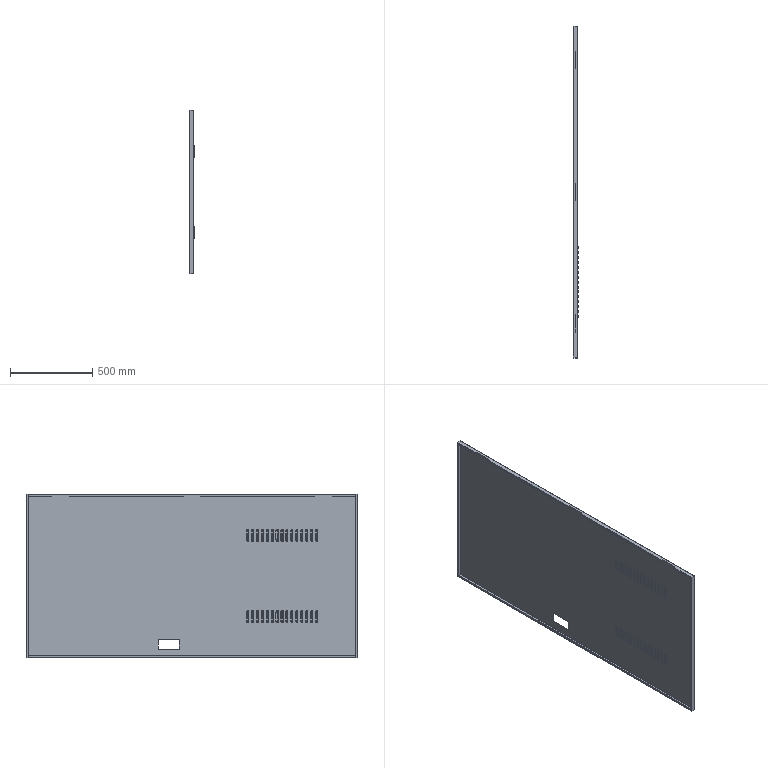Component | SolidWorks | SideDoorPanel-1 | 1 solid | 836 faces | volume 3311563 mm3 | cylinder 382 | torus 240 | plane 214 | commonest cylinder face diameters 8 x180 5 x90 11 x90 3.4 x11 0.4 x11